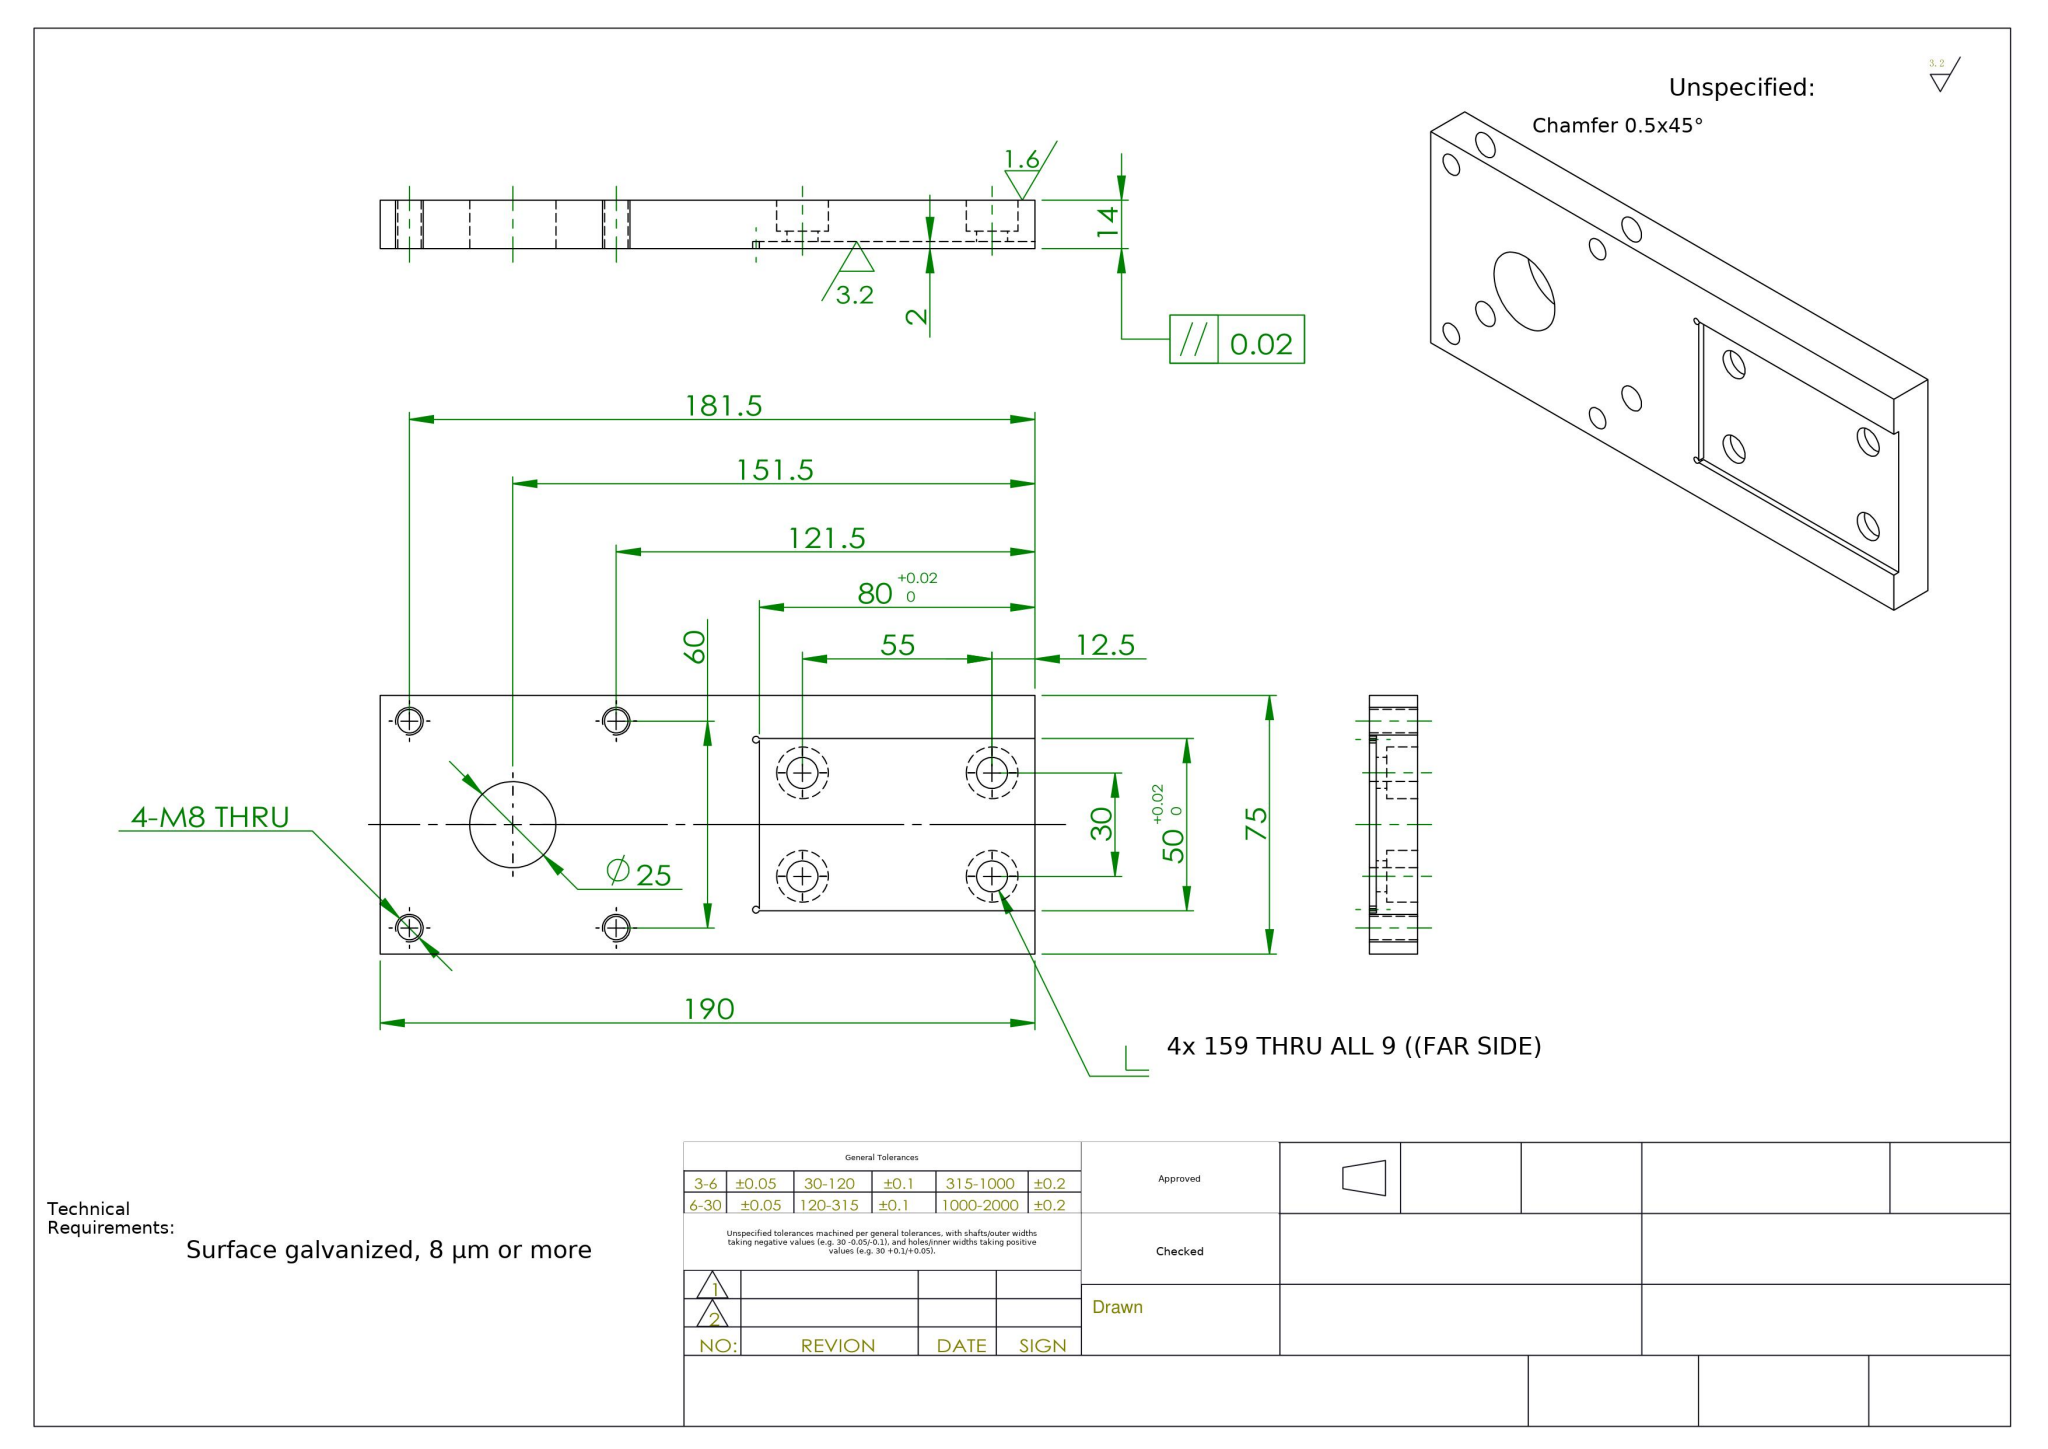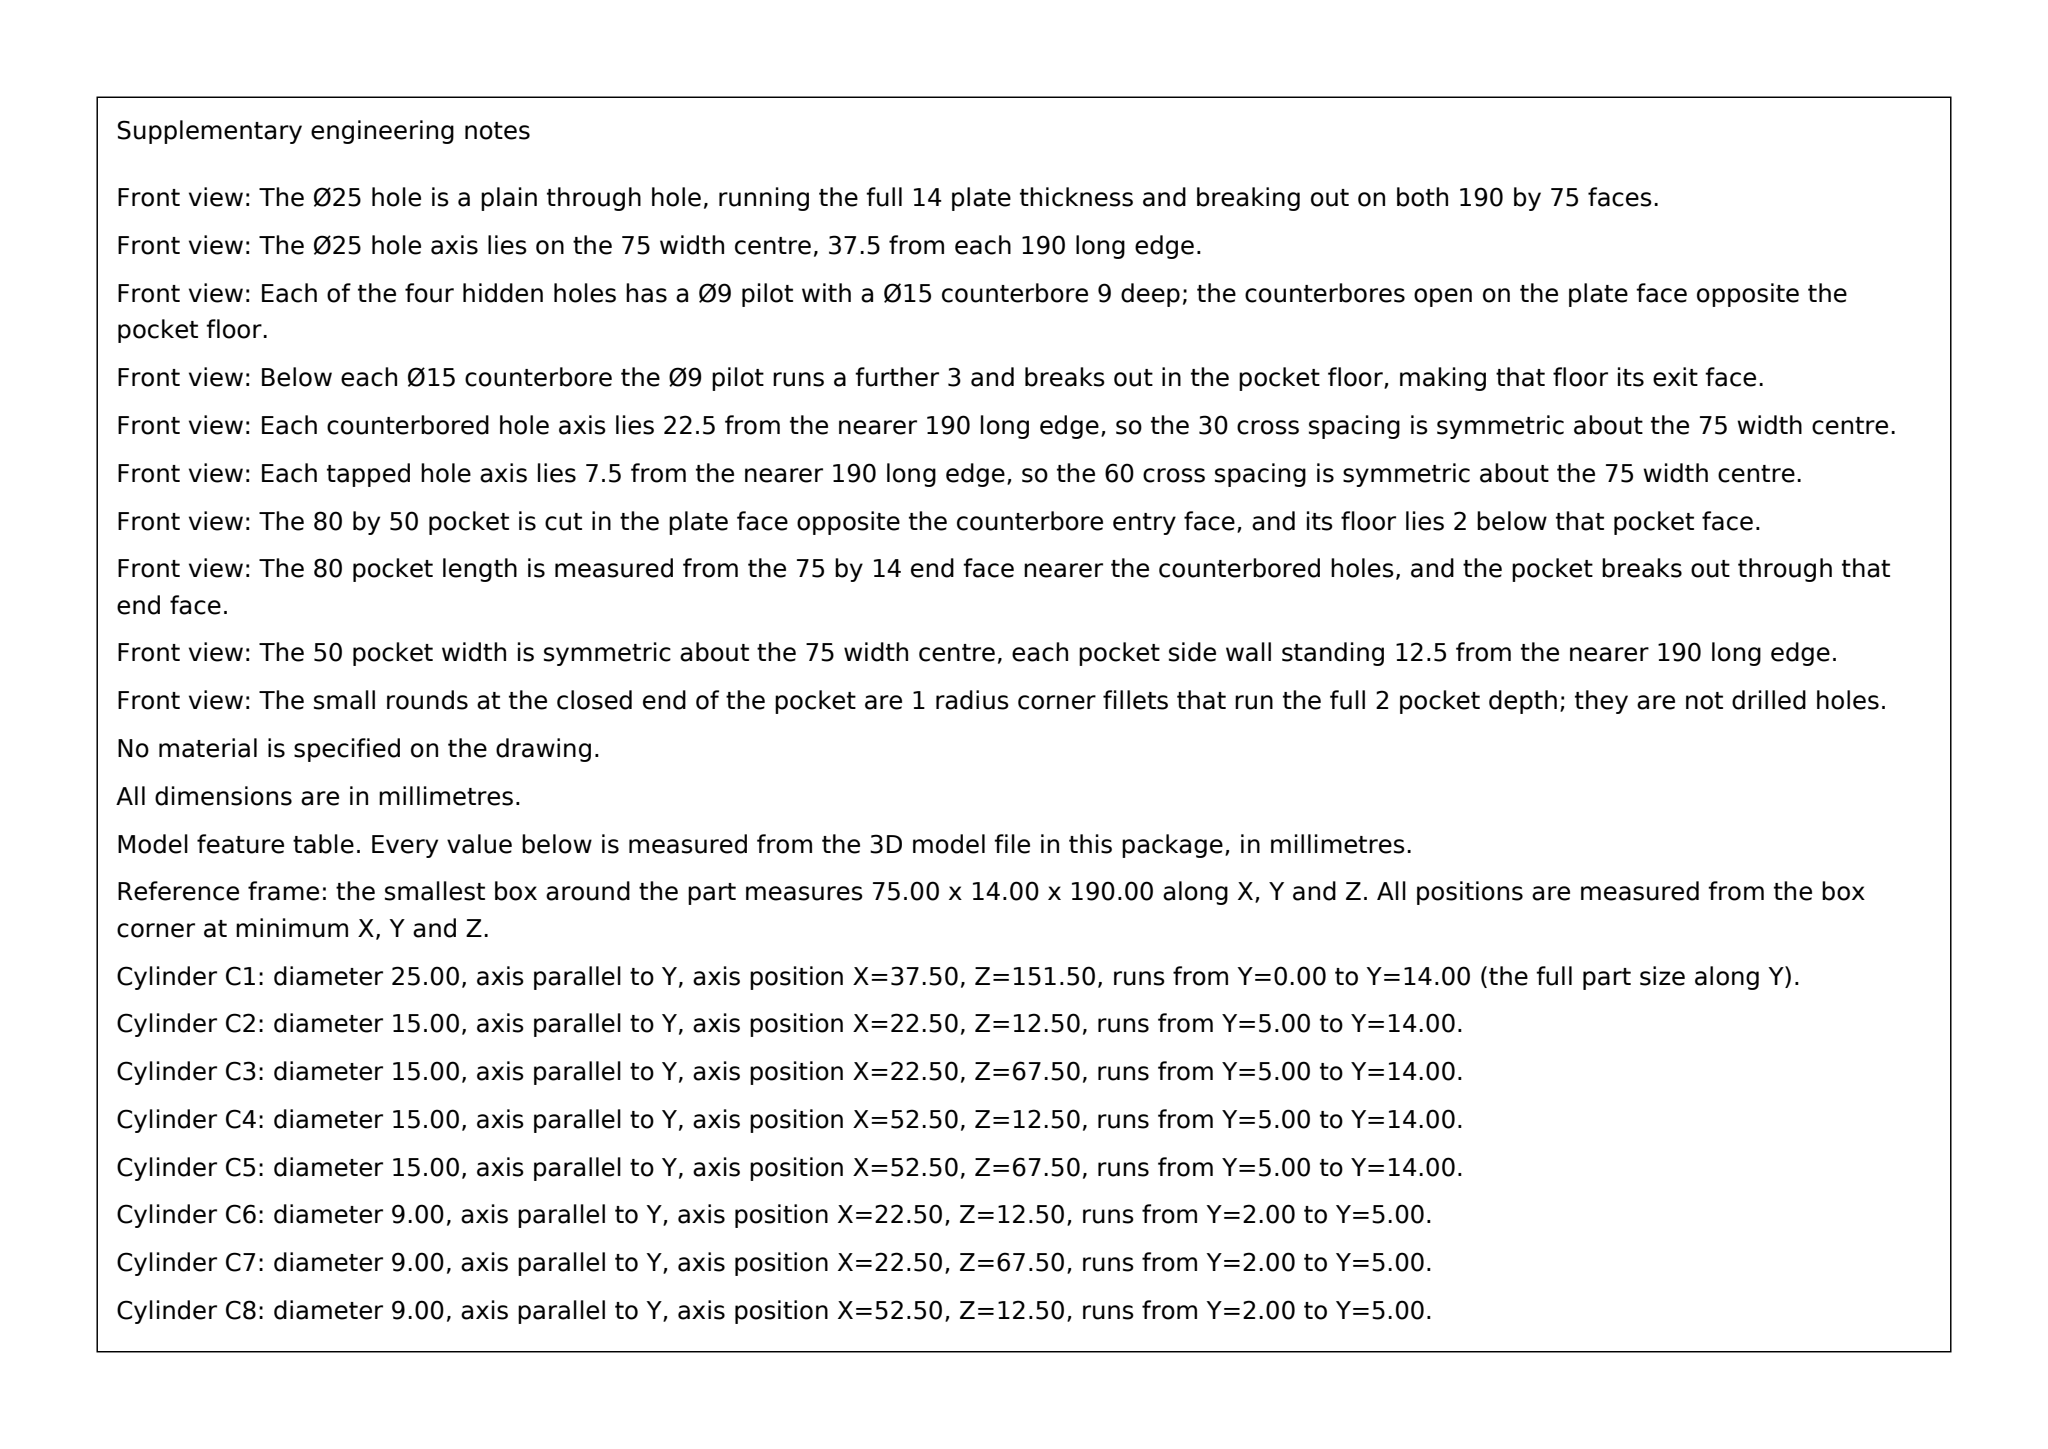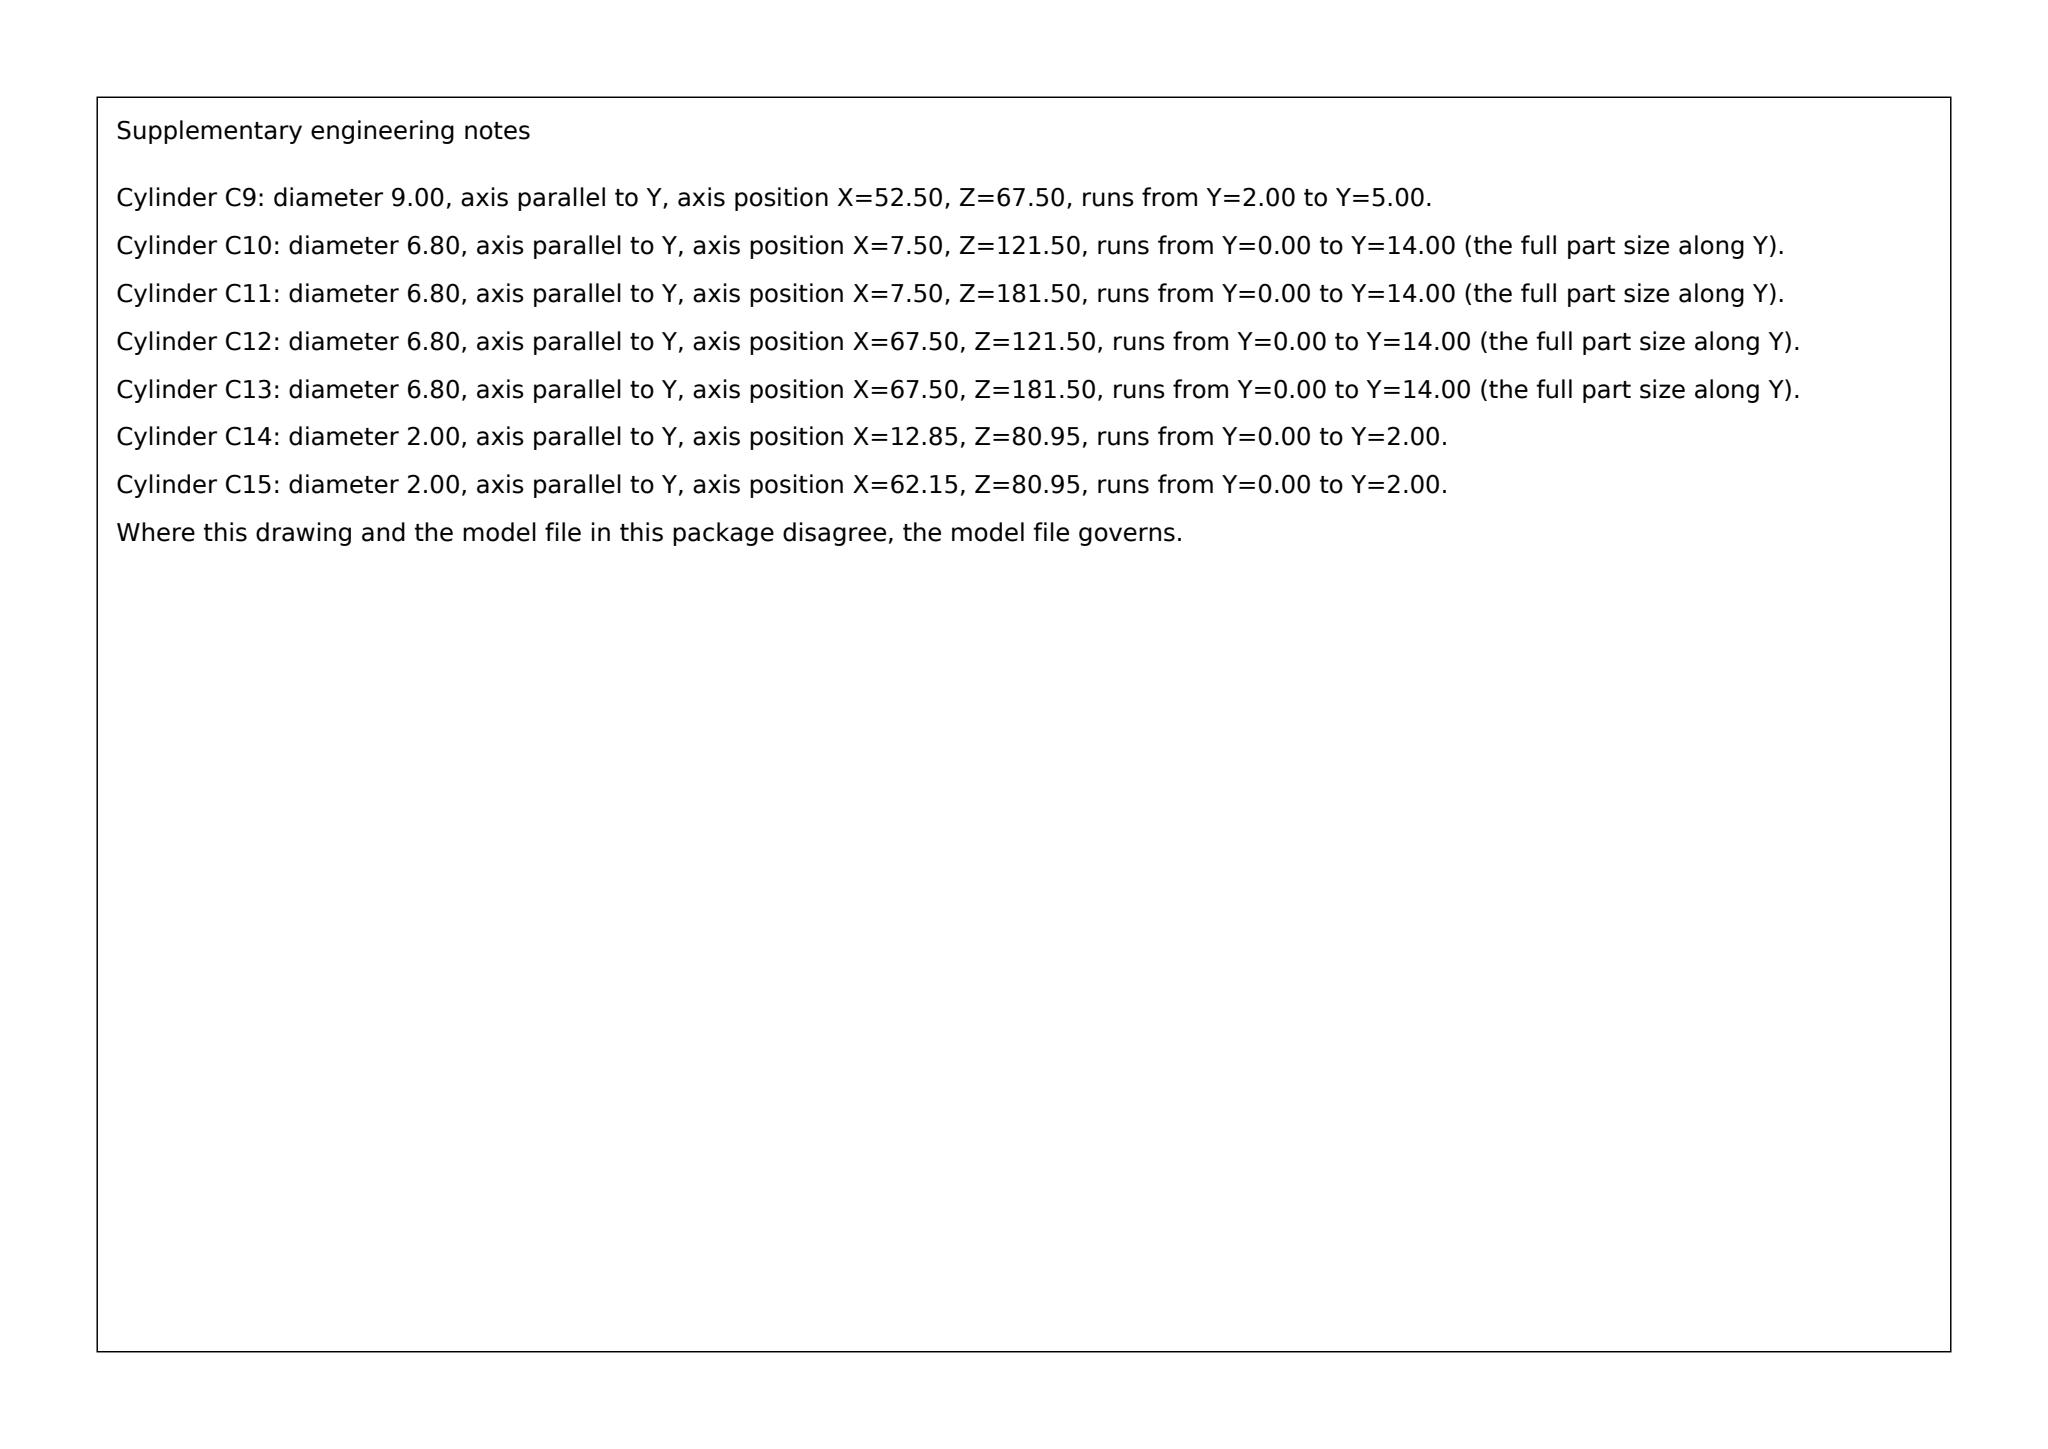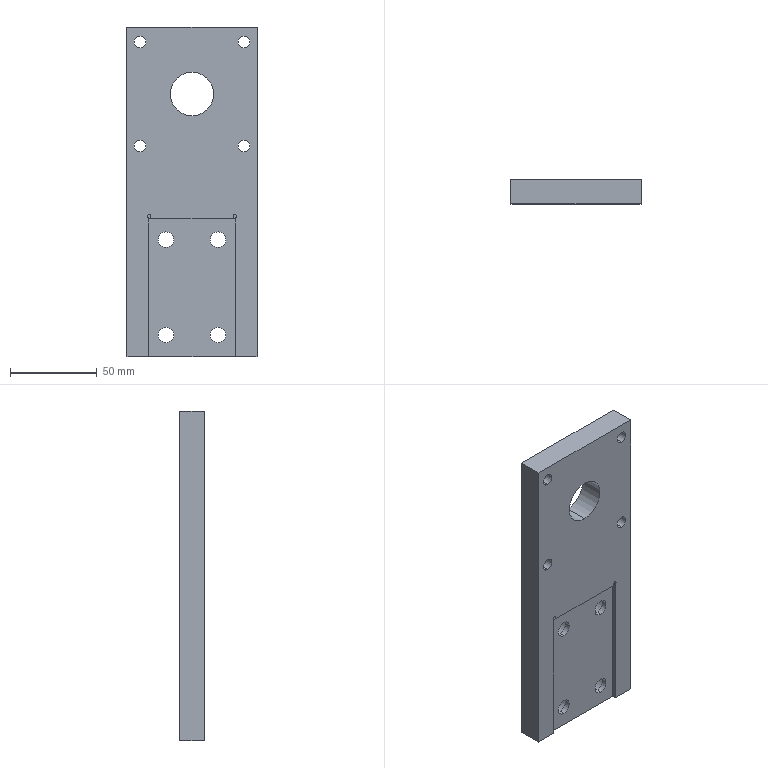Part | SolidWorks | mm | 1 solid | 42 faces | box 75 x 14 x 190 mm | volume 175456 mm3 | cylinder 28 | plane 14 | commonest cylinder face diameters 6.8 x8 9 x8 15 x8 25 x2 2 x2
Drawing notes:
4X Ø9 THRU ALL, CBORE Ø15 DP 9 FROM 14 FACE, BREAKS INTO 2 DP POCKET | from the solid: cyl Ø9 L3 and Ø15 L9 at x22.5/52.5, z12.5/67.5, y-axis; Ø15 from y=14 to y=5, Ø9 to pocket floor y=2
2X Ø2 DP 2, 80.95 FR RH END, 49.3 APART SYMM ABT CL | from the solid: Ø2 y-axis holes at (x12.85,z80.95) & (x62.15,z80.95), L2; 75 wide, CL=37.5
build123d program:
from build123d import *

# Parameters (mm, degrees)
SKETCH1_W                                       = 75
SKETCH1_H                                       = 190
EXTRUDE1_DEPTH                                  = 7
CUT_EXTRUDE1_DEPTH                              = 2
M8_HEX_SOCKET_HEAD_CAP_SCREW_CBORE1_D           = 9
M8_HEX_SOCKET_HEAD_CAP_SCREW_CBORE1_CBORE_D     = 15
M8_HEX_SOCKET_HEAD_CAP_SCREW_CBORE1_CBORE_DEPTH = 9
M8_TAPPED_HOLE1_D                               = 6.8
SKETCH7_R                                       = 12.5
CUT_EXTRUDE2_DEPTH                              = 104.089


with BuildPart() as part:
    # Sketch1 → Extrude1 (new, symmetric)
    with BuildSketch(Plane(origin=(0, 0, 0), x_dir=(1, 0, 0), z_dir=(0, 1, 0))):
        Rectangle(SKETCH1_W, SKETCH1_H)
    extrude(amount=EXTRUDE1_DEPTH, both=True)

    # Sketch2 → Cut-Extrude1 (cut)
    with BuildSketch(Plane.XZ.offset(7)):
        with BuildLine():
            Line((25, -95), (-25, -95))
            Line((-25, -95), (-25, -14.981))
            ThreePointArc((-25, -14.981), (-24.619, -13.045), (-24.352, -15))
            Line((-24.352, -15), (24.352, -15))
            ThreePointArc((24.352, -15), (24.619, -13.045), (25, -14.981))
            Line((25, -14.981), (25, -95))
        make_face()
    extrude(amount=-CUT_EXTRUDE1_DEPTH, mode=Mode.SUBTRACT)

    # M8 Hex Socket Head Cap Screw CBORE1 (through all)
    with Locations(Plane(origin=(0, 7, 0), x_dir=(-1, 0, 0), z_dir=(0, 1, 0))):
        with Locations((15, -82.5), (-15, -82.5), (-15, -27.5), (15, -27.5)):
            CounterBoreHole(M8_HEX_SOCKET_HEAD_CAP_SCREW_CBORE1_D / 2, M8_HEX_SOCKET_HEAD_CAP_SCREW_CBORE1_CBORE_D / 2, M8_HEX_SOCKET_HEAD_CAP_SCREW_CBORE1_CBORE_DEPTH)

    # M8 Tapped Hole1 (through all)
    with Locations(Plane(origin=(0, 7, 0), x_dir=(-1, 0, 0), z_dir=(0, 1, 0))):
        with Locations((30, 26.5), (-30, 26.5), (30, 86.5), (-30, 86.5)):
            Hole(M8_TAPPED_HOLE1_D / 2)

    # Sketch7 → Cut-Extrude2 (cut, through all)
    with BuildSketch(Plane(origin=(0, 7, 0), x_dir=(1, 0, 0), z_dir=(0, 1, 0))):
        with Locations(Location((0, -56.5, 0), (0, 0, 270))):
            Circle(SKETCH7_R)
    extrude(amount=-CUT_EXTRUDE2_DEPTH, mode=Mode.SUBTRACT)


solid = part.part